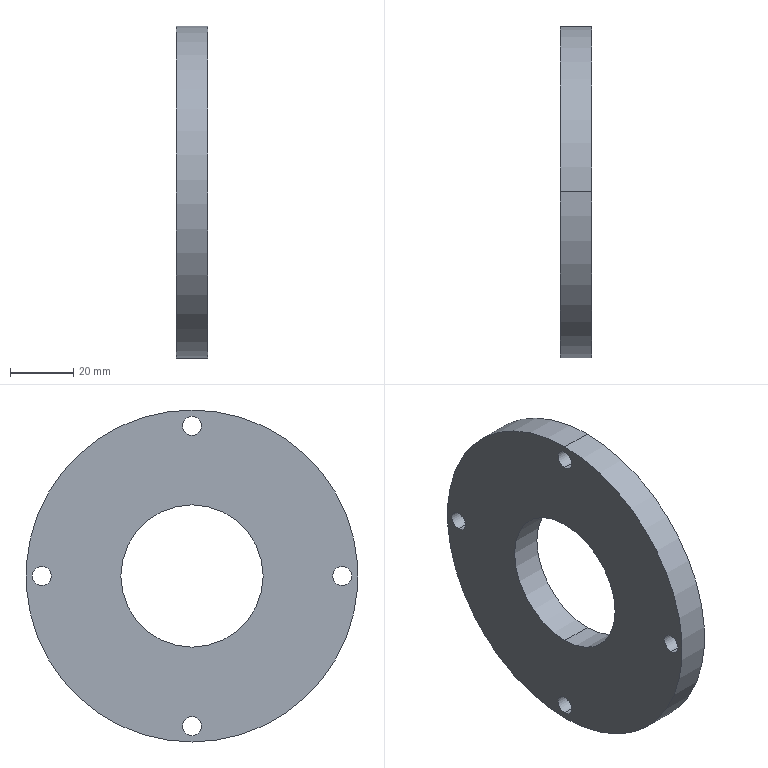Component | SolidWorks | Part10-1 | 1 solid | 22 faces | box 10 x 105 x 105 mm | volume 69545 mm3 | cylinder 12 | cone 8 | plane 2 | commonest cylinder face diameters 6 x8 45 x2 105 x2 | material ASTM A36 Steel
build123d program:
from build123d import *

# Parameters (mm, degrees)
SKETCH1_R           = 52.5
SKETCH1_R_2         = 3
SKETCH1_R_3         = 22.5
BOSS_EXTRUDE1_DEPTH = 10
CHAMFER1_SIZE       = 0.5


with BuildPart() as part:
    # Sketch1 → Boss-Extrude1 (new body)
    with BuildSketch(Plane.XY):
        Circle(SKETCH1_R)
        with Locations((-47.5, 0)):
            Circle(SKETCH1_R_2, mode=Mode.SUBTRACT)
        with Locations((0, -47.5)):
            Circle(SKETCH1_R_2, mode=Mode.SUBTRACT)
        with Locations((47.5, 0)):
            Circle(SKETCH1_R_2, mode=Mode.SUBTRACT)
        with Locations((0, 47.5)):
            Circle(SKETCH1_R_2, mode=Mode.SUBTRACT)
        Circle(SKETCH1_R_3, mode=Mode.SUBTRACT)
    extrude(amount=BOSS_EXTRUDE1_DEPTH)

    # Chamfer1
    chamfer1_edges = [part.edges().sort_by_distance(p)[0] for p in [
        (44.5, 0, 10),
        (-3, 47.5, 10),
        (-50.5, 0, 10),
        (-3, -47.5, 10),
    ]]
    chamfer(chamfer1_edges, length=CHAMFER1_SIZE)


solid = part.part

# Placed as in the assembly
solid = solid.moved(Location((37.5, -110, 40), (0, 90, 0)))
STEP:
#1=COLOUR_RGB('',0.7922,0.8196,0.9333);
#2=FILL_AREA_STYLE_COLOUR('',#1);
#3=FILL_AREA_STYLE('',(#2));
#4=SURFACE_STYLE_FILL_AREA(#3);
#5=SURFACE_SIDE_STYLE('',(#4));
#6=SURFACE_STYLE_USAGE(.BOTH.,#5);
#7=PRESENTATION_STYLE_ASSIGNMENT((#6));
#8=CARTESIAN_POINT('',(1.85,-4.331,3.563));
#9=VERTEX_POINT('',#8);
#10=CARTESIAN_POINT('',(1.85,-4.331,3.327));
#11=VERTEX_POINT('',#10);
#12=CARTESIAN_POINT('',(1.85,-4.331,3.445));
#13=DIRECTION('',(1.,0.,0.));
#14=DIRECTION('',(0.,0.,-1.));
#15=AXIS2_PLACEMENT_3D('',#12,#13,#14);
#16=CIRCLE('',#15,0.1181);
#17=EDGE_CURVE('',#9,#11,#16,.T.);
#18=ORIENTED_EDGE('',*,*,#17,.F.);
#19=CARTESIAN_POINT('',(1.87,-4.331,3.583));
#20=VERTEX_POINT('',#19);
#21=CARTESIAN_POINT('',(1.85,-4.331,3.563));
#22=DIRECTION('',(0.7071,0.,0.7071));
#23=VECTOR('',#22,39.37);
#24=LINE('',#21,#23);
#25=EDGE_CURVE('',#9,#20,#24,.T.);
#26=ORIENTED_EDGE('',*,*,#25,.T.);
#27=CARTESIAN_POINT('',(1.87,-4.331,3.307));
#28=VERTEX_POINT('',#27);
#29=CARTESIAN_POINT('',(1.87,-4.331,3.445));
#30=DIRECTION('',(-1.,0.,0.));
#31=DIRECTION('',(0.,0.,-1.));
#32=AXIS2_PLACEMENT_3D('',#29,#30,#31);
#33=CIRCLE('',#32,0.1378);
#34=EDGE_CURVE('',#28,#20,#33,.T.);
#35=ORIENTED_EDGE('',*,*,#34,.F.);
#36=CARTESIAN_POINT('',(1.85,-4.331,3.327));
#37=DIRECTION('',(0.7071,0.,-0.7071));
#38=VECTOR('',#37,39.37);
#39=LINE('',#36,#38);
#40=EDGE_CURVE('',#11,#28,#39,.T.);
#41=ORIENTED_EDGE('',*,*,#40,.F.);
#42=EDGE_LOOP('',(#18,#26,#35,#41));
#43=FACE_OUTER_BOUND('',#42,.T.);
#44=CARTESIAN_POINT('',(1.85,-4.331,3.445));
#45=DIRECTION('',(1.,0.,0.));
#46=DIRECTION('',(0.,0.,-1.));
#47=AXIS2_PLACEMENT_3D('',#44,#45,#46);
#48=CONICAL_SURFACE('',#47,0.1181,0.7854);
#49=ADVANCED_FACE('',(#43),#48,.F.);
#50=CARTESIAN_POINT('',(1.85,-6.201,1.693));
#51=VERTEX_POINT('',#50);
#52=CARTESIAN_POINT('',(1.85,-6.201,1.457));
#53=VERTEX_POINT('',#52);
#54=CARTESIAN_POINT('',(1.85,-6.201,1.575));
#55=DIRECTION('',(1.,0.,0.));
#56=DIRECTION('',(0.,0.,-1.));
#57=AXIS2_PLACEMENT_3D('',#54,#55,#56);
#58=CIRCLE('',#57,0.1181);
#59=EDGE_CURVE('',#51,#53,#58,.T.);
#60=ORIENTED_EDGE('',*,*,#59,.F.);
#61=CARTESIAN_POINT('',(1.87,-6.201,1.713));
#62=VERTEX_POINT('',#61);
#63=CARTESIAN_POINT('',(1.85,-6.201,1.693));
#64=DIRECTION('',(0.7071,0.,0.7071));
#65=VECTOR('',#64,39.37);
#66=LINE('',#63,#65);
#67=EDGE_CURVE('',#51,#62,#66,.T.);
#68=ORIENTED_EDGE('',*,*,#67,.T.);
#69=CARTESIAN_POINT('',(1.87,-6.201,1.437));
#70=VERTEX_POINT('',#69);
#71=CARTESIAN_POINT('',(1.87,-6.201,1.575));
#72=DIRECTION('',(-1.,0.,0.));
#73=DIRECTION('',(0.,0.,-1.));
#74=AXIS2_PLACEMENT_3D('',#71,#72,#73);
#75=CIRCLE('',#74,0.1378);
#76=EDGE_CURVE('',#70,#62,#75,.T.);
#77=ORIENTED_EDGE('',*,*,#76,.F.);
#78=CARTESIAN_POINT('',(1.85,-6.201,1.457));
#79=DIRECTION('',(0.7071,0.,-0.7071));
#80=VECTOR('',#79,39.37);
#81=LINE('',#78,#80);
#82=EDGE_CURVE('',#53,#70,#81,.T.);
#83=ORIENTED_EDGE('',*,*,#82,.F.);
#84=EDGE_LOOP('',(#60,#68,#77,#83));
#85=FACE_OUTER_BOUND('',#84,.T.);
#86=CARTESIAN_POINT('',(1.85,-6.201,1.575));
#87=DIRECTION('',(1.,0.,0.));
#88=DIRECTION('',(0.,0.,-1.));
#89=AXIS2_PLACEMENT_3D('',#86,#87,#88);
#90=CONICAL_SURFACE('',#89,0.1181,0.7854);
#91=ADVANCED_FACE('',(#85),#90,.F.);
#92=CARTESIAN_POINT('',(1.85,-4.331,-0.1772));
#93=VERTEX_POINT('',#92);
#94=CARTESIAN_POINT('',(1.85,-4.331,-0.4134));
#95=VERTEX_POINT('',#94);
#96=CARTESIAN_POINT('',(1.85,-4.331,-0.2953));
#97=DIRECTION('',(1.,0.,0.));
#98=DIRECTION('',(0.,0.,-1.));
#99=AXIS2_PLACEMENT_3D('',#96,#97,#98);
#100=CIRCLE('',#99,0.1181);
#101=EDGE_CURVE('',#93,#95,#100,.T.);
#102=ORIENTED_EDGE('',*,*,#101,.F.);
#103=CARTESIAN_POINT('',(1.87,-4.331,-0.1575));
#104=VERTEX_POINT('',#103);
#105=CARTESIAN_POINT('',(1.85,-4.331,-0.1772));
#106=DIRECTION('',(0.7071,0.,0.7071));
#107=VECTOR('',#106,39.37);
#108=LINE('',#105,#107);
#109=EDGE_CURVE('',#93,#104,#108,.T.);
#110=ORIENTED_EDGE('',*,*,#109,.T.);
#111=CARTESIAN_POINT('',(1.87,-4.331,-0.4331));
#112=VERTEX_POINT('',#111);
#113=CARTESIAN_POINT('',(1.87,-4.331,-0.2953));
#114=DIRECTION('',(-1.,0.,0.));
#115=DIRECTION('',(0.,0.,-1.));
#116=AXIS2_PLACEMENT_3D('',#113,#114,#115);
#117=CIRCLE('',#116,0.1378);
#118=EDGE_CURVE('',#112,#104,#117,.T.);
#119=ORIENTED_EDGE('',*,*,#118,.F.);
#120=CARTESIAN_POINT('',(1.85,-4.331,-0.4134));
#121=DIRECTION('',(0.7071,0.,-0.7071));
#122=VECTOR('',#121,39.37);
#123=LINE('',#120,#122);
#124=EDGE_CURVE('',#95,#112,#123,.T.);
#125=ORIENTED_EDGE('',*,*,#124,.F.);
#126=EDGE_LOOP('',(#102,#110,#119,#125));
#127=FACE_OUTER_BOUND('',#126,.T.);
#128=CARTESIAN_POINT('',(1.85,-4.331,-0.2953));
#129=DIRECTION('',(1.,0.,0.));
#130=DIRECTION('',(0.,0.,-1.));
#131=AXIS2_PLACEMENT_3D('',#128,#129,#130);
#132=CONICAL_SURFACE('',#131,0.1181,0.7854);
#133=ADVANCED_FACE('',(#127),#132,.F.);
#134=CARTESIAN_POINT('',(1.85,-2.461,1.693));
#135=VERTEX_POINT('',#134);
#136=CARTESIAN_POINT('',(1.85,-2.461,1.457));
#137=VERTEX_POINT('',#136);
#138=CARTESIAN_POINT('',(1.85,-2.461,1.575));
#139=DIRECTION('',(1.,0.,0.));
#140=DIRECTION('',(0.,0.,-1.));
#141=AXIS2_PLACEMENT_3D('',#138,#139,#140);
#142=CIRCLE('',#141,0.1181);
#143=EDGE_CURVE('',#135,#137,#142,.T.);
#144=ORIENTED_EDGE('',*,*,#143,.F.);
#145=CARTESIAN_POINT('',(1.87,-2.461,1.713));
#146=VERTEX_POINT('',#145);
#147=CARTESIAN_POINT('',(1.85,-2.461,1.693));
#148=DIRECTION('',(0.7071,0.,0.7071));
#149=VECTOR('',#148,39.37);
#150=LINE('',#147,#149);
#151=EDGE_CURVE('',#135,#146,#150,.T.);
#152=ORIENTED_EDGE('',*,*,#151,.T.);
#153=CARTESIAN_POINT('',(1.87,-2.461,1.437));
#154=VERTEX_POINT('',#153);
#155=CARTESIAN_POINT('',(1.87,-2.461,1.575));
#156=DIRECTION('',(-1.,0.,0.));
#157=DIRECTION('',(0.,0.,-1.));
#158=AXIS2_PLACEMENT_3D('',#155,#156,#157);
#159=CIRCLE('',#158,0.1378);
#160=EDGE_CURVE('',#154,#146,#159,.T.);
#161=ORIENTED_EDGE('',*,*,#160,.F.);
#162=CARTESIAN_POINT('',(1.85,-2.461,1.457));
#163=DIRECTION('',(0.7071,0.,-0.7071));
#164=VECTOR('',#163,39.37);
#165=LINE('',#162,#164);
#166=EDGE_CURVE('',#137,#154,#165,.T.);
#167=ORIENTED_EDGE('',*,*,#166,.F.);
#168=EDGE_LOOP('',(#144,#152,#161,#167));
#169=FACE_OUTER_BOUND('',#168,.T.);
#170=CARTESIAN_POINT('',(1.85,-2.461,1.575));
#171=DIRECTION('',(1.,0.,0.));
#172=DIRECTION('',(0.,0.,-1.));
#173=AXIS2_PLACEMENT_3D('',#170,#171,#172);
#174=CONICAL_SURFACE('',#173,0.1181,0.7854);
#175=ADVANCED_FACE('',(#169),#174,.F.);
#176=CARTESIAN_POINT('',(1.87,-4.331,2.461));
#177=VERTEX_POINT('',#176);
#178=CARTESIAN_POINT('',(1.87,-4.331,0.689));
#179=VERTEX_POINT('',#178);
#180=CARTESIAN_POINT('',(1.87,-4.331,1.575));
#181=DIRECTION('',(1.,0.,0.));
#182=DIRECTION('',(0.,0.,-1.));
#183=AXIS2_PLACEMENT_3D('',#180,#181,#182);
#184=CIRCLE('',#183,0.8858);
#185=EDGE_CURVE('',#177,#179,#184,.T.);
#186=ORIENTED_EDGE('',*,*,#185,.T.);
#187=CARTESIAN_POINT('',(1.476,-4.331,0.689));
#188=VERTEX_POINT('',#187);
#189=CARTESIAN_POINT('',(1.87,-4.331,0.689));
#190=DIRECTION('',(-1.,0.,0.));
#191=VECTOR('',#190,39.37);
#192=LINE('',#189,#191);
#193=EDGE_CURVE('',#179,#188,#192,.T.);
#194=ORIENTED_EDGE('',*,*,#193,.T.);
#195=CARTESIAN_POINT('',(1.476,-4.331,2.461));
#196=VERTEX_POINT('',#195);
#197=CARTESIAN_POINT('',(1.476,-4.331,1.575));
#198=DIRECTION('',(1.,0.,0.));
#199=DIRECTION('',(0.,0.,-1.));
#200=AXIS2_PLACEMENT_3D('',#197,#198,#199);
#201=CIRCLE('',#200,0.8858);
#202=EDGE_CURVE('',#196,#188,#201,.T.);
#203=ORIENTED_EDGE('',*,*,#202,.F.);
#204=CARTESIAN_POINT('',(1.87,-4.331,2.461));
#205=DIRECTION('',(-1.,0.,0.));
#206=VECTOR('',#205,39.37);
#207=LINE('',#204,#206);
#208=EDGE_CURVE('',#177,#196,#207,.T.);
#209=ORIENTED_EDGE('',*,*,#208,.F.);
#210=EDGE_LOOP('',(#186,#194,#203,#209));
#211=FACE_OUTER_BOUND('',#210,.T.);
#212=CARTESIAN_POINT('',(1.87,-4.331,1.575));
#213=DIRECTION('',(-1.,0.,0.));
#214=DIRECTION('',(0.,0.,1.));
#215=AXIS2_PLACEMENT_3D('',#212,#213,#214);
#216=CYLINDRICAL_SURFACE('',#215,0.8858);
#217=ADVANCED_FACE('',(#211),#216,.F.);
#218=ORIENTED_EDGE('',*,*,#143,.T.);
#219=CARTESIAN_POINT('',(1.476,-2.461,1.457));
#220=VERTEX_POINT('',#219);
#221=CARTESIAN_POINT('',(1.87,-2.461,1.457));
#222=DIRECTION('',(-1.,0.,0.));
#223=VECTOR('',#222,39.37);
#224=LINE('',#221,#223);
#225=EDGE_CURVE('',#137,#220,#224,.T.);
#226=ORIENTED_EDGE('',*,*,#225,.T.);
#227=CARTESIAN_POINT('',(1.476,-2.461,1.693));
#228=VERTEX_POINT('',#227);
#229=CARTESIAN_POINT('',(1.476,-2.461,1.575));
#230=DIRECTION('',(1.,0.,0.));
#231=DIRECTION('',(0.,0.,-1.));
#232=AXIS2_PLACEMENT_3D('',#229,#230,#231);
#233=CIRCLE('',#232,0.1181);
#234=EDGE_CURVE('',#228,#220,#233,.T.);
#235=ORIENTED_EDGE('',*,*,#234,.F.);
#236=CARTESIAN_POINT('',(1.87,-2.461,1.693));
#237=DIRECTION('',(-1.,0.,0.));
#238=VECTOR('',#237,39.37);
#239=LINE('',#236,#238);
#240=EDGE_CURVE('',#135,#228,#239,.T.);
#241=ORIENTED_EDGE('',*,*,#240,.F.);
#242=EDGE_LOOP('',(#218,#226,#235,#241));
#243=FACE_OUTER_BOUND('',#242,.T.);
#244=CARTESIAN_POINT('',(1.87,-2.461,1.575));
#245=DIRECTION('',(-1.,0.,0.));
#246=DIRECTION('',(0.,0.,1.));
#247=AXIS2_PLACEMENT_3D('',#244,#245,#246);
#248=CYLINDRICAL_SURFACE('',#247,0.1181);
#249=ADVANCED_FACE('',(#243),#248,.F.);
#250=ORIENTED_EDGE('',*,*,#101,.T.);
#251=CARTESIAN_POINT('',(1.476,-4.331,-0.4134));
#252=VERTEX_POINT('',#251);
#253=CARTESIAN_POINT('',(1.87,-4.331,-0.4134));
#254=DIRECTION('',(-1.,0.,0.));
#255=VECTOR('',#254,39.37);
#256=LINE('',#253,#255);
#257=EDGE_CURVE('',#95,#252,#256,.T.);
#258=ORIENTED_EDGE('',*,*,#257,.T.);
#259=CARTESIAN_POINT('',(1.476,-4.331,-0.1772));
#260=VERTEX_POINT('',#259);
#261=CARTESIAN_POINT('',(1.476,-4.331,-0.2953));
#262=DIRECTION('',(1.,0.,0.));
#263=DIRECTION('',(0.,0.,-1.));
#264=AXIS2_PLACEMENT_3D('',#261,#262,#263);
#265=CIRCLE('',#264,0.1181);
#266=EDGE_CURVE('',#260,#252,#265,.T.);
#267=ORIENTED_EDGE('',*,*,#266,.F.);
#268=CARTESIAN_POINT('',(1.87,-4.331,-0.1772));
#269=DIRECTION('',(-1.,0.,0.));
#270=VECTOR('',#269,39.37);
#271=LINE('',#268,#270);
#272=EDGE_CURVE('',#93,#260,#271,.T.);
#273=ORIENTED_EDGE('',*,*,#272,.F.);
#274=EDGE_LOOP('',(#250,#258,#267,#273));
#275=FACE_OUTER_BOUND('',#274,.T.);
#276=CARTESIAN_POINT('',(1.87,-4.331,-0.2953));
#277=DIRECTION('',(-1.,0.,0.));
#278=DIRECTION('',(0.,0.,1.));
#279=AXIS2_PLACEMENT_3D('',#276,#277,#278);
#280=CYLINDRICAL_SURFACE('',#279,0.1181);
#281=ADVANCED_FACE('',(#275),#280,.F.);
#282=ORIENTED_EDGE('',*,*,#59,.T.);
#283=CARTESIAN_POINT('',(1.476,-6.201,1.457));
#284=VERTEX_POINT('',#283);
#285=CARTESIAN_POINT('',(1.87,-6.201,1.457));
#286=DIRECTION('',(-1.,0.,0.));
#287=VECTOR('',#286,39.37);
#288=LINE('',#285,#287);
#289=EDGE_CURVE('',#53,#284,#288,.T.);
#290=ORIENTED_EDGE('',*,*,#289,.T.);
#291=CARTESIAN_POINT('',(1.476,-6.201,1.693));
#292=VERTEX_POINT('',#291);
#293=CARTESIAN_POINT('',(1.476,-6.201,1.575));
#294=DIRECTION('',(1.,0.,0.));
#295=DIRECTION('',(0.,0.,-1.));
#296=AXIS2_PLACEMENT_3D('',#293,#294,#295);
#297=CIRCLE('',#296,0.1181);
#298=EDGE_CURVE('',#292,#284,#297,.T.);
#299=ORIENTED_EDGE('',*,*,#298,.F.);
#300=CARTESIAN_POINT('',(1.87,-6.201,1.693));
#301=DIRECTION('',(-1.,0.,0.));
#302=VECTOR('',#301,39.37);
#303=LINE('',#300,#302);
#304=EDGE_CURVE('',#51,#292,#303,.T.);
#305=ORIENTED_EDGE('',*,*,#304,.F.);
#306=EDGE_LOOP('',(#282,#290,#299,#305));
#307=FACE_OUTER_BOUND('',#306,.T.);
#308=CARTESIAN_POINT('',(1.87,-6.201,1.575));
#309=DIRECTION('',(-1.,0.,0.));
#310=DIRECTION('',(0.,0.,1.));
#311=AXIS2_PLACEMENT_3D('',#308,#309,#310);
#312=CYLINDRICAL_SURFACE('',#311,0.1181);
#313=ADVANCED_FACE('',(#307),#312,.F.);
#314=ORIENTED_EDGE('',*,*,#17,.T.);
#315=CARTESIAN_POINT('',(1.476,-4.331,3.327));
#316=VERTEX_POINT('',#315);
#317=CARTESIAN_POINT('',(1.87,-4.331,3.327));
#318=DIRECTION('',(-1.,0.,0.));
#319=VECTOR('',#318,39.37);
#320=LINE('',#317,#319);
#321=EDGE_CURVE('',#11,#316,#320,.T.);
#322=ORIENTED_EDGE('',*,*,#321,.T.);
#323=CARTESIAN_POINT('',(1.476,-4.331,3.563));
#324=VERTEX_POINT('',#323);
#325=CARTESIAN_POINT('',(1.476,-4.331,3.445));
#326=DIRECTION('',(1.,0.,0.));
#327=DIRECTION('',(0.,0.,-1.));
#328=AXIS2_PLACEMENT_3D('',#325,#326,#327);
#329=CIRCLE('',#328,0.1181);
#330=EDGE_CURVE('',#324,#316,#329,.T.);
#331=ORIENTED_EDGE('',*,*,#330,.F.);
#332=CARTESIAN_POINT('',(1.87,-4.331,3.563));
#333=DIRECTION('',(-1.,0.,0.));
#334=VECTOR('',#333,39.37);
#335=LINE('',#332,#334);
#336=EDGE_CURVE('',#9,#324,#335,.T.);
#337=ORIENTED_EDGE('',*,*,#336,.F.);
#338=EDGE_LOOP('',(#314,#322,#331,#337));
#339=FACE_OUTER_BOUND('',#338,.T.);
#340=CARTESIAN_POINT('',(1.87,-4.331,3.445));
#341=DIRECTION('',(-1.,0.,0.));
#342=DIRECTION('',(0.,0.,1.));
#343=AXIS2_PLACEMENT_3D('',#340,#341,#342);
#344=CYLINDRICAL_SURFACE('',#343,0.1181);
#345=ADVANCED_FACE('',(#339),#344,.F.);
#346=CARTESIAN_POINT('',(1.87,-4.331,-0.4921));
#347=VERTEX_POINT('',#346);
#348=CARTESIAN_POINT('',(1.87,-4.331,3.642));
#349=VERTEX_POINT('',#348);
#350=CARTESIAN_POINT('',(1.87,-4.331,1.575));
#351=DIRECTION('',(1.,0.,0.));
#352=DIRECTION('',(0.,0.,-1.));
#353=AXIS2_PLACEMENT_3D('',#350,#351,#352);
#354=CIRCLE('',#353,2.067);
#355=EDGE_CURVE('',#347,#349,#354,.T.);
#356=ORIENTED_EDGE('',*,*,#355,.F.);
#357=CARTESIAN_POINT('',(1.476,-4.331,-0.4921));
#358=VERTEX_POINT('',#357);
#359=CARTESIAN_POINT('',(1.87,-4.331,-0.4921));
#360=DIRECTION('',(-1.,0.,0.));
#361=VECTOR('',#360,39.37);
#362=LINE('',#359,#361);
#363=EDGE_CURVE('',#347,#358,#362,.T.);
#364=ORIENTED_EDGE('',*,*,#363,.T.);
#365=CARTESIAN_POINT('',(1.476,-4.331,3.642));
#366=VERTEX_POINT('',#365);
#367=CARTESIAN_POINT('',(1.476,-4.331,1.575));
#368=DIRECTION('',(1.,0.,0.));
#369=DIRECTION('',(0.,0.,-1.));
#370=AXIS2_PLACEMENT_3D('',#367,#368,#369);
#371=CIRCLE('',#370,2.067);
#372=EDGE_CURVE('',#358,#366,#371,.T.);
#373=ORIENTED_EDGE('',*,*,#372,.T.);
#374=CARTESIAN_POINT('',(1.87,-4.331,3.642));
#375=DIRECTION('',(-1.,0.,0.));
#376=VECTOR('',#375,39.37);
#377=LINE('',#374,#376);
#378=EDGE_CURVE('',#349,#366,#377,.T.);
#379=ORIENTED_EDGE('',*,*,#378,.F.);
#380=EDGE_LOOP('',(#356,#364,#373,#379));
#381=FACE_OUTER_BOUND('',#380,.T.);
#382=CARTESIAN_POINT('',(1.87,-4.331,1.575));
#383=DIRECTION('',(-1.,0.,0.));
#384=DIRECTION('',(0.,0.,1.));
#385=AXIS2_PLACEMENT_3D('',#382,#383,#384);
#386=CYLINDRICAL_SURFACE('',#385,2.067);
#387=ADVANCED_FACE('',(#381),#386,.T.);
#388=ORIENTED_EDGE('',*,*,#160,.T.);
#389=CARTESIAN_POINT('',(1.87,-2.461,1.575));
#390=DIRECTION('',(-1.,0.,0.));
#391=DIRECTION('',(0.,0.,-1.));
#392=AXIS2_PLACEMENT_3D('',#389,#390,#391);
#393=CIRCLE('',#392,0.1378);
#394=EDGE_CURVE('',#146,#154,#393,.T.);
#395=ORIENTED_EDGE('',*,*,#394,.T.);
#396=EDGE_LOOP('',(#388,#395));
#397=FACE_BOUND('',#396,.T.);
#398=ORIENTED_EDGE('',*,*,#118,.T.);
#399=CARTESIAN_POINT('',(1.87,-4.331,-0.2953));
#400=DIRECTION('',(-1.,0.,0.));
#401=DIRECTION('',(0.,0.,-1.));
#402=AXIS2_PLACEMENT_3D('',#399,#400,#401);
#403=CIRCLE('',#402,0.1378);
#404=EDGE_CURVE('',#104,#112,#403,.T.);
#405=ORIENTED_EDGE('',*,*,#404,.T.);
#406=EDGE_LOOP('',(#398,#405));
#407=FACE_BOUND('',#406,.T.);
#408=ORIENTED_EDGE('',*,*,#76,.T.);
#409=CARTESIAN_POINT('',(1.87,-6.201,1.575));
#410=DIRECTION('',(-1.,0.,0.));
#411=DIRECTION('',(0.,0.,-1.));
#412=AXIS2_PLACEMENT_3D('',#409,#410,#411);
#413=CIRCLE('',#412,0.1378);
#414=EDGE_CURVE('',#62,#70,#413,.T.);
#415=ORIENTED_EDGE('',*,*,#414,.T.);
#416=EDGE_LOOP('',(#408,#415));
#417=FACE_BOUND('',#416,.T.);
#418=ORIENTED_EDGE('',*,*,#34,.T.);
#419=CARTESIAN_POINT('',(1.87,-4.331,3.445));
#420=DIRECTION('',(-1.,0.,0.));
#421=DIRECTION('',(0.,0.,-1.));
#422=AXIS2_PLACEMENT_3D('',#419,#420,#421);
#423=CIRCLE('',#422,0.1378);
#424=EDGE_CURVE('',#20,#28,#423,.T.);
#425=ORIENTED_EDGE('',*,*,#424,.T.);
#426=EDGE_LOOP('',(#418,#425));
#427=FACE_BOUND('',#426,.T.);
#428=CARTESIAN_POINT('',(1.87,-4.331,1.575));
#429=DIRECTION('',(1.,0.,0.));
#430=DIRECTION('',(0.,0.,-1.));
#431=AXIS2_PLACEMENT_3D('',#428,#429,#430);
#432=CIRCLE('',#431,2.067);
#433=EDGE_CURVE('',#349,#347,#432,.T.);
#434=ORIENTED_EDGE('',*,*,#433,.T.);
#435=ORIENTED_EDGE('',*,*,#355,.T.);
#436=EDGE_LOOP('',(#434,#435));
#437=FACE_OUTER_BOUND('',#436,.T.);
#438=ORIENTED_EDGE('',*,*,#185,.F.);
#439=CARTESIAN_POINT('',(1.87,-4.331,1.575));
#440=DIRECTION('',(1.,0.,0.));
#441=DIRECTION('',(0.,0.,-1.));
#442=AXIS2_PLACEMENT_3D('',#439,#440,#441);
#443=CIRCLE('',#442,0.8858);
#444=EDGE_CURVE('',#179,#177,#443,.T.);
#445=ORIENTED_EDGE('',*,*,#444,.F.);
#446=EDGE_LOOP('',(#438,#445));
#447=FACE_BOUND('',#446,.T.);
#448=CARTESIAN_POINT('',(1.87,-4.331,1.575));
#449=DIRECTION('',(1.,0.,0.));
#450=DIRECTION('',(0.,0.,-1.));
#451=AXIS2_PLACEMENT_3D('',#448,#449,#450);
#452=PLANE('',#451);
#453=ADVANCED_FACE('',(#397,#407,#417,#427,#437,#447),#452,.T.);
#454=CARTESIAN_POINT('',(1.476,-4.331,1.575));
#455=DIRECTION('',(1.,0.,0.));
#456=DIRECTION('',(0.,0.,-1.));
#457=AXIS2_PLACEMENT_3D('',#454,#455,#456);
#458=CIRCLE('',#457,2.067);
#459=EDGE_CURVE('',#366,#358,#458,.T.);
#460=ORIENTED_EDGE('',*,*,#459,.F.);
#461=ORIENTED_EDGE('',*,*,#372,.F.);
#462=EDGE_LOOP('',(#460,#461));
#463=FACE_OUTER_BOUND('',#462,.T.);
#464=ORIENTED_EDGE('',*,*,#330,.T.);
#465=CARTESIAN_POINT('',(1.476,-4.331,3.445));
#466=DIRECTION('',(1.,0.,0.));
#467=DIRECTION('',(0.,0.,-1.));
#468=AXIS2_PLACEMENT_3D('',#465,#466,#467);
#469=CIRCLE('',#468,0.1181);
#470=EDGE_CURVE('',#316,#324,#469,.T.);
#471=ORIENTED_EDGE('',*,*,#470,.T.);
#472=EDGE_LOOP('',(#464,#471));
#473=FACE_BOUND('',#472,.T.);
#474=ORIENTED_EDGE('',*,*,#298,.T.);
#475=CARTESIAN_POINT('',(1.476,-6.201,1.575));
#476=DIRECTION('',(1.,0.,0.));
#477=DIRECTION('',(0.,0.,-1.));
#478=AXIS2_PLACEMENT_3D('',#475,#476,#477);
#479=CIRCLE('',#478,0.1181);
#480=EDGE_CURVE('',#284,#292,#479,.T.);
#481=ORIENTED_EDGE('',*,*,#480,.T.);
#482=EDGE_LOOP('',(#474,#481));
#483=FACE_BOUND('',#482,.T.);
#484=ORIENTED_EDGE('',*,*,#266,.T.);
#485=CARTESIAN_POINT('',(1.476,-4.331,-0.2953));
#486=DIRECTION('',(1.,0.,0.));
#487=DIRECTION('',(0.,0.,-1.));
#488=AXIS2_PLACEMENT_3D('',#485,#486,#487);
#489=CIRCLE('',#488,0.1181);
#490=EDGE_CURVE('',#252,#260,#489,.T.);
#491=ORIENTED_EDGE('',*,*,#490,.T.);
#492=EDGE_LOOP('',(#484,#491));
#493=FACE_BOUND('',#492,.T.);
#494=ORIENTED_EDGE('',*,*,#234,.T.);
#495=CARTESIAN_POINT('',(1.476,-2.461,1.575));
#496=DIRECTION('',(1.,0.,0.));
#497=DIRECTION('',(0.,0.,-1.));
#498=AXIS2_PLACEMENT_3D('',#495,#496,#497);
#499=CIRCLE('',#498,0.1181);
#500=EDGE_CURVE('',#220,#228,#499,.T.);
#501=ORIENTED_EDGE('',*,*,#500,.T.);
#502=EDGE_LOOP('',(#494,#501));
#503=FACE_BOUND('',#502,.T.);
#504=ORIENTED_EDGE('',*,*,#202,.T.);
#505=CARTESIAN_POINT('',(1.476,-4.331,1.575));
#506=DIRECTION('',(1.,0.,0.));
#507=DIRECTION('',(0.,0.,-1.));
#508=AXIS2_PLACEMENT_3D('',#505,#506,#507);
#509=CIRCLE('',#508,0.8858);
#510=EDGE_CURVE('',#188,#196,#509,.T.);
#511=ORIENTED_EDGE('',*,*,#510,.T.);
#512=EDGE_LOOP('',(#504,#511));
#513=FACE_BOUND('',#512,.T.);
#514=CARTESIAN_POINT('',(1.476,-4.331,1.575));
#515=DIRECTION('',(1.,0.,0.));
#516=DIRECTION('',(0.,0.,-1.));
#517=AXIS2_PLACEMENT_3D('',#514,#515,#516);
#518=PLANE('',#517);
#519=ADVANCED_FACE('',(#463,#473,#483,#493,#503,#513),#518,.F.);
#520=ORIENTED_EDGE('',*,*,#363,.F.);
#521=ORIENTED_EDGE('',*,*,#433,.F.);
#522=ORIENTED_EDGE('',*,*,#378,.T.);
#523=ORIENTED_EDGE('',*,*,#459,.T.);
#524=EDGE_LOOP('',(#520,#521,#522,#523));
#525=FACE_OUTER_BOUND('',#524,.T.);
#526=CARTESIAN_POINT('',(1.87,-4.331,1.575));
#527=DIRECTION('',(-1.,0.,0.));
#528=DIRECTION('',(0.,0.,1.));
#529=AXIS2_PLACEMENT_3D('',#526,#527,#528);
#530=CYLINDRICAL_SURFACE('',#529,2.067);
#531=ADVANCED_FACE('',(#525),#530,.T.);
#532=ORIENTED_EDGE('',*,*,#321,.F.);
#533=CARTESIAN_POINT('',(1.85,-4.331,3.445));
#534=DIRECTION('',(1.,0.,0.));
#535=DIRECTION('',(0.,0.,-1.));
#536=AXIS2_PLACEMENT_3D('',#533,#534,#535);
#537=CIRCLE('',#536,0.1181);
#538=EDGE_CURVE('',#11,#9,#537,.T.);
#539=ORIENTED_EDGE('',*,*,#538,.T.);
#540=ORIENTED_EDGE('',*,*,#336,.T.);
#541=ORIENTED_EDGE('',*,*,#470,.F.);
#542=EDGE_LOOP('',(#532,#539,#540,#541));
#543=FACE_OUTER_BOUND('',#542,.T.);
#544=CARTESIAN_POINT('',(1.87,-4.331,3.445));
#545=DIRECTION('',(-1.,0.,0.));
#546=DIRECTION('',(0.,0.,1.));
#547=AXIS2_PLACEMENT_3D('',#544,#545,#546);
#548=CYLINDRICAL_SURFACE('',#547,0.1181);
#549=ADVANCED_FACE('',(#543),#548,.F.);
#550=ORIENTED_EDGE('',*,*,#289,.F.);
#551=CARTESIAN_POINT('',(1.85,-6.201,1.575));
#552=DIRECTION('',(1.,0.,0.));
#553=DIRECTION('',(0.,0.,-1.));
#554=AXIS2_PLACEMENT_3D('',#551,#552,#553);
#555=CIRCLE('',#554,0.1181);
#556=EDGE_CURVE('',#53,#51,#555,.T.);
#557=ORIENTED_EDGE('',*,*,#556,.T.);
#558=ORIENTED_EDGE('',*,*,#304,.T.);
#559=ORIENTED_EDGE('',*,*,#480,.F.);
#560=EDGE_LOOP('',(#550,#557,#558,#559));
#561=FACE_OUTER_BOUND('',#560,.T.);
#562=CARTESIAN_POINT('',(1.87,-6.201,1.575));
#563=DIRECTION('',(-1.,0.,0.));
#564=DIRECTION('',(0.,0.,1.));
#565=AXIS2_PLACEMENT_3D('',#562,#563,#564);
#566=CYLINDRICAL_SURFACE('',#565,0.1181);
#567=ADVANCED_FACE('',(#561),#566,.F.);
#568=ORIENTED_EDGE('',*,*,#257,.F.);
#569=CARTESIAN_POINT('',(1.85,-4.331,-0.2953));
#570=DIRECTION('',(1.,0.,0.));
#571=DIRECTION('',(0.,0.,-1.));
#572=AXIS2_PLACEMENT_3D('',#569,#570,#571);
#573=CIRCLE('',#572,0.1181);
#574=EDGE_CURVE('',#95,#93,#573,.T.);
#575=ORIENTED_EDGE('',*,*,#574,.T.);
#576=ORIENTED_EDGE('',*,*,#272,.T.);
#577=ORIENTED_EDGE('',*,*,#490,.F.);
#578=EDGE_LOOP('',(#568,#575,#576,#577));
#579=FACE_OUTER_BOUND('',#578,.T.);
#580=CARTESIAN_POINT('',(1.87,-4.331,-0.2953));
#581=DIRECTION('',(-1.,0.,0.));
#582=DIRECTION('',(0.,0.,1.));
#583=AXIS2_PLACEMENT_3D('',#580,#581,#582);
#584=CYLINDRICAL_SURFACE('',#583,0.1181);
#585=ADVANCED_FACE('',(#579),#584,.F.);
#586=ORIENTED_EDGE('',*,*,#225,.F.);
#587=CARTESIAN_POINT('',(1.85,-2.461,1.575));
#588=DIRECTION('',(1.,0.,0.));
#589=DIRECTION('',(0.,0.,-1.));
#590=AXIS2_PLACEMENT_3D('',#587,#588,#589);
#591=CIRCLE('',#590,0.1181);
#592=EDGE_CURVE('',#137,#135,#591,.T.);
#593=ORIENTED_EDGE('',*,*,#592,.T.);
#594=ORIENTED_EDGE('',*,*,#240,.T.);
#595=ORIENTED_EDGE('',*,*,#500,.F.);
#596=EDGE_LOOP('',(#586,#593,#594,#595));
#597=FACE_OUTER_BOUND('',#596,.T.);
#598=CARTESIAN_POINT('',(1.87,-2.461,1.575));
#599=DIRECTION('',(-1.,0.,0.));
#600=DIRECTION('',(0.,0.,1.));
#601=AXIS2_PLACEMENT_3D('',#598,#599,#600);
#602=CYLINDRICAL_SURFACE('',#601,0.1181);
#603=ADVANCED_FACE('',(#597),#602,.F.);
#604=ORIENTED_EDGE('',*,*,#193,.F.);
#605=ORIENTED_EDGE('',*,*,#444,.T.);
#606=ORIENTED_EDGE('',*,*,#208,.T.);
#607=ORIENTED_EDGE('',*,*,#510,.F.);
#608=EDGE_LOOP('',(#604,#605,#606,#607));
#609=FACE_OUTER_BOUND('',#608,.T.);
#610=CARTESIAN_POINT('',(1.87,-4.331,1.575));
#611=DIRECTION('',(-1.,0.,0.));
#612=DIRECTION('',(0.,0.,1.));
#613=AXIS2_PLACEMENT_3D('',#610,#611,#612);
#614=CYLINDRICAL_SURFACE('',#613,0.8858);
#615=ADVANCED_FACE('',(#609),#614,.F.);
#616=ORIENTED_EDGE('',*,*,#151,.F.);
#617=ORIENTED_EDGE('',*,*,#592,.F.);
#618=ORIENTED_EDGE('',*,*,#166,.T.);
#619=ORIENTED_EDGE('',*,*,#394,.F.);
#620=EDGE_LOOP('',(#616,#617,#618,#619));
#621=FACE_OUTER_BOUND('',#620,.T.);
#622=CARTESIAN_POINT('',(1.85,-2.461,1.575));
#623=DIRECTION('',(1.,0.,0.));
#624=DIRECTION('',(0.,0.,-1.));
#625=AXIS2_PLACEMENT_3D('',#622,#623,#624);
#626=CONICAL_SURFACE('',#625,0.1181,0.7854);
#627=ADVANCED_FACE('',(#621),#626,.F.);
#628=ORIENTED_EDGE('',*,*,#109,.F.);
#629=ORIENTED_EDGE('',*,*,#574,.F.);
#630=ORIENTED_EDGE('',*,*,#124,.T.);
#631=ORIENTED_EDGE('',*,*,#404,.F.);
#632=EDGE_LOOP('',(#628,#629,#630,#631));
#633=FACE_OUTER_BOUND('',#632,.T.);
#634=CARTESIAN_POINT('',(1.85,-4.331,-0.2953));
#635=DIRECTION('',(1.,0.,0.));
#636=DIRECTION('',(0.,0.,-1.));
#637=AXIS2_PLACEMENT_3D('',#634,#635,#636);
#638=CONICAL_SURFACE('',#637,0.1181,0.7854);
#639=ADVANCED_FACE('',(#633),#638,.F.);
#640=ORIENTED_EDGE('',*,*,#67,.F.);
#641=ORIENTED_EDGE('',*,*,#556,.F.);
#642=ORIENTED_EDGE('',*,*,#82,.T.);
#643=ORIENTED_EDGE('',*,*,#414,.F.);
#644=EDGE_LOOP('',(#640,#641,#642,#643));
#645=FACE_OUTER_BOUND('',#644,.T.);
#646=CARTESIAN_POINT('',(1.85,-6.201,1.575));
#647=DIRECTION('',(1.,0.,0.));
#648=DIRECTION('',(0.,0.,-1.));
#649=AXIS2_PLACEMENT_3D('',#646,#647,#648);
#650=CONICAL_SURFACE('',#649,0.1181,0.7854);
#651=ADVANCED_FACE('',(#645),#650,.F.);
#652=ORIENTED_EDGE('',*,*,#25,.F.);
#653=ORIENTED_EDGE('',*,*,#538,.F.);
#654=ORIENTED_EDGE('',*,*,#40,.T.);
#655=ORIENTED_EDGE('',*,*,#424,.F.);
#656=EDGE_LOOP('',(#652,#653,#654,#655));
#657=FACE_OUTER_BOUND('',#656,.T.);
#658=CARTESIAN_POINT('',(1.85,-4.331,3.445));
#659=DIRECTION('',(1.,0.,0.));
#660=DIRECTION('',(0.,0.,-1.));
#661=AXIS2_PLACEMENT_3D('',#658,#659,#660);
#662=CONICAL_SURFACE('',#661,0.1181,0.7854);
#663=ADVANCED_FACE('',(#657),#662,.F.);
#664=CLOSED_SHELL('',(#49,#91,#133,#175,#217,#249,#281,#313,#345,#387,#453,#519,#531,#549,#567,#585,#603,#615,#627,#639,#651,#663));
#665=MANIFOLD_SOLID_BREP('',#664);
#666=STYLED_ITEM('',(#7),#665);
#667=PRESENTATION_LAYER_ASSIGNMENT('','',(#666));
#668=CARTESIAN_POINT('',(0.,0.,0.));
#669=DIRECTION('',(0.,0.,1.));
#670=DIRECTION('',(1.,0.,0.));
#671=AXIS2_PLACEMENT_3D('',#668,#669,#670);
#672=(LENGTH_UNIT()NAMED_UNIT(*)SI_UNIT($,.METRE.));
#673=LENGTH_MEASURE_WITH_UNIT(LENGTH_MEASURE(0.0254),#672);
#674=DIMENSIONAL_EXPONENTS(1.,0.,0.,0.,0.,0.,0.);
#675=(CONVERSION_BASED_UNIT('',#673)LENGTH_UNIT()NAMED_UNIT(#674));
#676=UNCERTAINTY_MEASURE_WITH_UNIT(LENGTH_MEASURE(0.00001),#675,'','');
#677=(NAMED_UNIT(*)PLANE_ANGLE_UNIT()SI_UNIT($,.RADIAN.));
#678=(NAMED_UNIT(*)SI_UNIT($,.STERADIAN.)SOLID_ANGLE_UNIT());
#679=(GEOMETRIC_REPRESENTATION_CONTEXT(3)GLOBAL_UNCERTAINTY_ASSIGNED_CONTEXT((#676))GLOBAL_UNIT_ASSIGNED_CONTEXT((#675,#677,#678))REPRESENTATION_CONTEXT('',''));
#680=ADVANCED_BREP_SHAPE_REPRESENTATION('',(#665,#671),#679);
#681=(LENGTH_UNIT()NAMED_UNIT(*)SI_UNIT($,.METRE.));
#682=LENGTH_MEASURE_WITH_UNIT(LENGTH_MEASURE(0.0254),#681);
#683=DIMENSIONAL_EXPONENTS(1.,0.,0.,0.,0.,0.,0.);
#684=(CONVERSION_BASED_UNIT('',#682)LENGTH_UNIT()NAMED_UNIT(#683));
#685=UNCERTAINTY_MEASURE_WITH_UNIT(LENGTH_MEASURE(0.00001),#684,'','');
#686=(NAMED_UNIT(*)PLANE_ANGLE_UNIT()SI_UNIT($,.RADIAN.));
#687=(NAMED_UNIT(*)SI_UNIT($,.STERADIAN.)SOLID_ANGLE_UNIT());
#688=(GEOMETRIC_REPRESENTATION_CONTEXT(3)GLOBAL_UNCERTAINTY_ASSIGNED_CONTEXT((#685))GLOBAL_UNIT_ASSIGNED_CONTEXT((#684,#686,#687))REPRESENTATION_CONTEXT('',''));
#689=MECHANICAL_DESIGN_GEOMETRIC_PRESENTATION_REPRESENTATION('',(#666),#688);